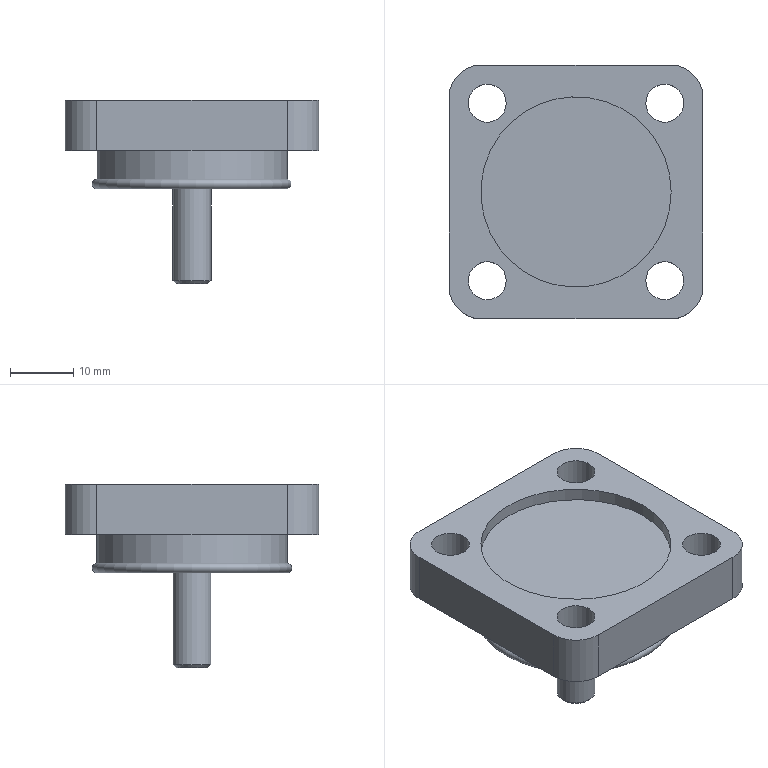Component | NX | UNI_WHEEL_BASE_2 | 2 solids | 23 faces | volume 15058 mm3 | cylinder 12 | plane 9 | torus 1 | cone 1 | commonest cylinder face diameters 6 x5 10 x4 30 x3